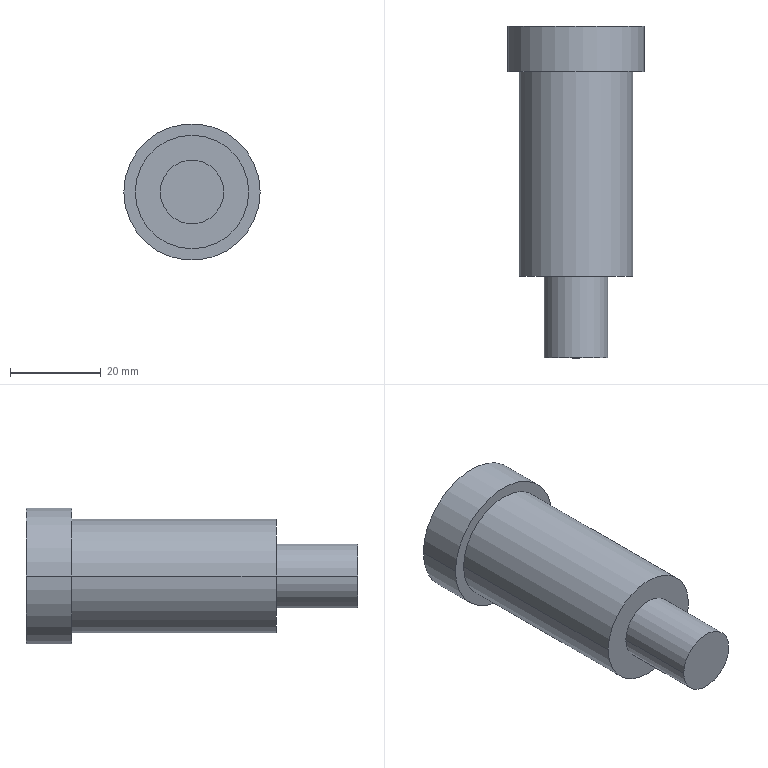Component | SolidWorks | FlipAxis-4 | 1 solid | 10 faces | box 30 x 73 x 30 mm | volume 31929 mm3 | cylinder 6 | plane 4 | commonest cylinder face diameters 14 x2 25 x2 30 x2 | material Plain Carbon Steel
build123d program:
from build123d import *

# Parameters (mm, degrees)
SKETCH1_R           = 15
BOSS_EXTRUDE1_DEPTH = 10
SKETCH2_R           = 12.5
BOSS_EXTRUDE2_DEPTH = 45
SKETCH3_R           = 7
BOSS_EXTRUDE3_DEPTH = 18


with BuildPart() as part:
    # Sketch1 → Boss-Extrude1 (new body)
    with BuildSketch(Plane.XY):
        Circle(SKETCH1_R)
    extrude(amount=BOSS_EXTRUDE1_DEPTH)

    # Sketch2 → Boss-Extrude2 (add)
    with BuildSketch(Plane.XY.offset(10)):
        with Locations(Location((0, 0, 0), (0, 0, 180))):
            Circle(SKETCH2_R)
    extrude(amount=BOSS_EXTRUDE2_DEPTH)

    # Sketch3 → Boss-Extrude3 (add)
    with BuildSketch(Plane.XY.offset(55)):
        Circle(SKETCH3_R)
    extrude(amount=BOSS_EXTRUDE3_DEPTH)


solid = part.part

# Placed as in the assembly
solid = solid.moved(Location((-864.885, -397.907, 1035.102), (90, 0, 0)))
STEP:
#1=COLOUR_RGB('',0.7922,0.8196,0.9333);
#2=FILL_AREA_STYLE_COLOUR('',#1);
#3=FILL_AREA_STYLE('',(#2));
#4=SURFACE_STYLE_FILL_AREA(#3);
#5=SURFACE_SIDE_STYLE('',(#4));
#6=SURFACE_STYLE_USAGE(.BOTH.,#5);
#7=PRESENTATION_STYLE_ASSIGNMENT((#6));
#8=CARTESIAN_POINT('',(-33.775,-18.54,40.752));
#9=VERTEX_POINT('',#8);
#10=CARTESIAN_POINT('',(-34.326,-18.54,40.752));
#11=VERTEX_POINT('',#10);
#12=CARTESIAN_POINT('',(-34.051,-18.54,40.752));
#13=DIRECTION('',(0.,-1.,0.));
#14=DIRECTION('',(1.,0.,0.));
#15=AXIS2_PLACEMENT_3D('',#12,#13,#14);
#16=CIRCLE('',#15,0.2756);
#17=EDGE_CURVE('',#9,#11,#16,.T.);
#18=ORIENTED_EDGE('',*,*,#17,.F.);
#19=CARTESIAN_POINT('',(-33.775,-17.831,40.752));
#20=VERTEX_POINT('',#19);
#21=CARTESIAN_POINT('',(-33.775,-18.54,40.752));
#22=DIRECTION('',(0.,1.,0.));
#23=VECTOR('',#22,39.37);
#24=LINE('',#21,#23);
#25=EDGE_CURVE('',#9,#20,#24,.T.);
#26=ORIENTED_EDGE('',*,*,#25,.T.);
#27=CARTESIAN_POINT('',(-34.326,-17.831,40.752));
#28=VERTEX_POINT('',#27);
#29=CARTESIAN_POINT('',(-34.051,-17.831,40.752));
#30=DIRECTION('',(0.,-1.,0.));
#31=DIRECTION('',(1.,0.,0.));
#32=AXIS2_PLACEMENT_3D('',#29,#30,#31);
#33=CIRCLE('',#32,0.2756);
#34=EDGE_CURVE('',#20,#28,#33,.T.);
#35=ORIENTED_EDGE('',*,*,#34,.T.);
#36=CARTESIAN_POINT('',(-34.326,-18.54,40.752));
#37=DIRECTION('',(0.,1.,0.));
#38=VECTOR('',#37,39.37);
#39=LINE('',#36,#38);
#40=EDGE_CURVE('',#11,#28,#39,.T.);
#41=ORIENTED_EDGE('',*,*,#40,.F.);
#42=EDGE_LOOP('',(#18,#26,#35,#41));
#43=FACE_OUTER_BOUND('',#42,.T.);
#44=CARTESIAN_POINT('',(-34.051,-18.54,40.752));
#45=DIRECTION('',(0.,1.,0.));
#46=DIRECTION('',(-1.,0.,0.));
#47=AXIS2_PLACEMENT_3D('',#44,#45,#46);
#48=CYLINDRICAL_SURFACE('',#47,0.2756);
#49=ADVANCED_FACE('',(#43),#48,.T.);
#50=CARTESIAN_POINT('',(-33.558,-17.831,40.752));
#51=VERTEX_POINT('',#50);
#52=CARTESIAN_POINT('',(-34.543,-17.831,40.752));
#53=VERTEX_POINT('',#52);
#54=CARTESIAN_POINT('',(-34.051,-17.831,40.752));
#55=DIRECTION('',(0.,-1.,0.));
#56=DIRECTION('',(1.,0.,0.));
#57=AXIS2_PLACEMENT_3D('',#54,#55,#56);
#58=CIRCLE('',#57,0.4921);
#59=EDGE_CURVE('',#51,#53,#58,.T.);
#60=ORIENTED_EDGE('',*,*,#59,.F.);
#61=CARTESIAN_POINT('',(-33.558,-16.059,40.752));
#62=VERTEX_POINT('',#61);
#63=CARTESIAN_POINT('',(-33.558,-17.831,40.752));
#64=DIRECTION('',(0.,1.,0.));
#65=VECTOR('',#64,39.37);
#66=LINE('',#63,#65);
#67=EDGE_CURVE('',#51,#62,#66,.T.);
#68=ORIENTED_EDGE('',*,*,#67,.T.);
#69=CARTESIAN_POINT('',(-34.543,-16.059,40.752));
#70=VERTEX_POINT('',#69);
#71=CARTESIAN_POINT('',(-34.051,-16.059,40.752));
#72=DIRECTION('',(0.,-1.,0.));
#73=DIRECTION('',(1.,0.,0.));
#74=AXIS2_PLACEMENT_3D('',#71,#72,#73);
#75=CIRCLE('',#74,0.4921);
#76=EDGE_CURVE('',#62,#70,#75,.T.);
#77=ORIENTED_EDGE('',*,*,#76,.T.);
#78=CARTESIAN_POINT('',(-34.543,-17.831,40.752));
#79=DIRECTION('',(0.,1.,0.));
#80=VECTOR('',#79,39.37);
#81=LINE('',#78,#80);
#82=EDGE_CURVE('',#53,#70,#81,.T.);
#83=ORIENTED_EDGE('',*,*,#82,.F.);
#84=EDGE_LOOP('',(#60,#68,#77,#83));
#85=FACE_OUTER_BOUND('',#84,.T.);
#86=CARTESIAN_POINT('',(-34.051,-17.831,40.752));
#87=DIRECTION('',(0.,1.,0.));
#88=DIRECTION('',(-1.,0.,0.));
#89=AXIS2_PLACEMENT_3D('',#86,#87,#88);
#90=CYLINDRICAL_SURFACE('',#89,0.4921);
#91=ADVANCED_FACE('',(#85),#90,.T.);
#92=CARTESIAN_POINT('',(-33.46,-16.059,40.752));
#93=VERTEX_POINT('',#92);
#94=CARTESIAN_POINT('',(-34.641,-16.059,40.752));
#95=VERTEX_POINT('',#94);
#96=CARTESIAN_POINT('',(-34.051,-16.059,40.752));
#97=DIRECTION('',(0.,-1.,0.));
#98=DIRECTION('',(1.,0.,0.));
#99=AXIS2_PLACEMENT_3D('',#96,#97,#98);
#100=CIRCLE('',#99,0.5906);
#101=EDGE_CURVE('',#93,#95,#100,.T.);
#102=ORIENTED_EDGE('',*,*,#101,.F.);
#103=CARTESIAN_POINT('',(-33.46,-15.666,40.752));
#104=VERTEX_POINT('',#103);
#105=CARTESIAN_POINT('',(-33.46,-16.059,40.752));
#106=DIRECTION('',(0.,1.,0.));
#107=VECTOR('',#106,39.37);
#108=LINE('',#105,#107);
#109=EDGE_CURVE('',#93,#104,#108,.T.);
#110=ORIENTED_EDGE('',*,*,#109,.T.);
#111=CARTESIAN_POINT('',(-34.641,-15.666,40.752));
#112=VERTEX_POINT('',#111);
#113=CARTESIAN_POINT('',(-34.051,-15.666,40.752));
#114=DIRECTION('',(0.,-1.,0.));
#115=DIRECTION('',(1.,0.,0.));
#116=AXIS2_PLACEMENT_3D('',#113,#114,#115);
#117=CIRCLE('',#116,0.5906);
#118=EDGE_CURVE('',#104,#112,#117,.T.);
#119=ORIENTED_EDGE('',*,*,#118,.T.);
#120=CARTESIAN_POINT('',(-34.641,-16.059,40.752));
#121=DIRECTION('',(0.,1.,0.));
#122=VECTOR('',#121,39.37);
#123=LINE('',#120,#122);
#124=EDGE_CURVE('',#95,#112,#123,.T.);
#125=ORIENTED_EDGE('',*,*,#124,.F.);
#126=EDGE_LOOP('',(#102,#110,#119,#125));
#127=FACE_OUTER_BOUND('',#126,.T.);
#128=CARTESIAN_POINT('',(-34.051,-16.059,40.752));
#129=DIRECTION('',(0.,1.,0.));
#130=DIRECTION('',(-1.,0.,0.));
#131=AXIS2_PLACEMENT_3D('',#128,#129,#130);
#132=CYLINDRICAL_SURFACE('',#131,0.5906);
#133=ADVANCED_FACE('',(#127),#132,.T.);
#134=CARTESIAN_POINT('',(-34.051,-17.831,40.752));
#135=DIRECTION('',(0.,-1.,0.));
#136=DIRECTION('',(1.,0.,0.));
#137=AXIS2_PLACEMENT_3D('',#134,#135,#136);
#138=CIRCLE('',#137,0.4921);
#139=EDGE_CURVE('',#53,#51,#138,.T.);
#140=ORIENTED_EDGE('',*,*,#139,.T.);
#141=ORIENTED_EDGE('',*,*,#59,.T.);
#142=EDGE_LOOP('',(#140,#141));
#143=FACE_OUTER_BOUND('',#142,.T.);
#144=CARTESIAN_POINT('',(-34.051,-17.831,40.752));
#145=DIRECTION('',(0.,-1.,0.));
#146=DIRECTION('',(1.,0.,0.));
#147=AXIS2_PLACEMENT_3D('',#144,#145,#146);
#148=CIRCLE('',#147,0.2756);
#149=EDGE_CURVE('',#28,#20,#148,.T.);
#150=ORIENTED_EDGE('',*,*,#149,.F.);
#151=ORIENTED_EDGE('',*,*,#34,.F.);
#152=EDGE_LOOP('',(#150,#151));
#153=FACE_BOUND('',#152,.T.);
#154=CARTESIAN_POINT('',(-34.051,-17.831,40.752));
#155=DIRECTION('',(0.,-1.,0.));
#156=DIRECTION('',(1.,0.,0.));
#157=AXIS2_PLACEMENT_3D('',#154,#155,#156);
#158=PLANE('',#157);
#159=ADVANCED_FACE('',(#143,#153),#158,.T.);
#160=CARTESIAN_POINT('',(-34.051,-16.059,40.752));
#161=DIRECTION('',(0.,-1.,0.));
#162=DIRECTION('',(1.,0.,0.));
#163=AXIS2_PLACEMENT_3D('',#160,#161,#162);
#164=CIRCLE('',#163,0.5906);
#165=EDGE_CURVE('',#95,#93,#164,.T.);
#166=ORIENTED_EDGE('',*,*,#165,.T.);
#167=ORIENTED_EDGE('',*,*,#101,.T.);
#168=EDGE_LOOP('',(#166,#167));
#169=FACE_OUTER_BOUND('',#168,.T.);
#170=CARTESIAN_POINT('',(-34.051,-16.059,40.752));
#171=DIRECTION('',(0.,-1.,0.));
#172=DIRECTION('',(1.,0.,0.));
#173=AXIS2_PLACEMENT_3D('',#170,#171,#172);
#174=CIRCLE('',#173,0.4921);
#175=EDGE_CURVE('',#70,#62,#174,.T.);
#176=ORIENTED_EDGE('',*,*,#175,.F.);
#177=ORIENTED_EDGE('',*,*,#76,.F.);
#178=EDGE_LOOP('',(#176,#177));
#179=FACE_BOUND('',#178,.T.);
#180=CARTESIAN_POINT('',(-34.051,-16.059,40.752));
#181=DIRECTION('',(0.,-1.,0.));
#182=DIRECTION('',(1.,0.,0.));
#183=AXIS2_PLACEMENT_3D('',#180,#181,#182);
#184=PLANE('',#183);
#185=ADVANCED_FACE('',(#169,#179),#184,.T.);
#186=ORIENTED_EDGE('',*,*,#109,.F.);
#187=ORIENTED_EDGE('',*,*,#165,.F.);
#188=ORIENTED_EDGE('',*,*,#124,.T.);
#189=CARTESIAN_POINT('',(-34.051,-15.666,40.752));
#190=DIRECTION('',(0.,-1.,0.));
#191=DIRECTION('',(1.,0.,0.));
#192=AXIS2_PLACEMENT_3D('',#189,#190,#191);
#193=CIRCLE('',#192,0.5906);
#194=EDGE_CURVE('',#112,#104,#193,.T.);
#195=ORIENTED_EDGE('',*,*,#194,.T.);
#196=EDGE_LOOP('',(#186,#187,#188,#195));
#197=FACE_OUTER_BOUND('',#196,.T.);
#198=CARTESIAN_POINT('',(-34.051,-16.059,40.752));
#199=DIRECTION('',(0.,1.,0.));
#200=DIRECTION('',(-1.,0.,0.));
#201=AXIS2_PLACEMENT_3D('',#198,#199,#200);
#202=CYLINDRICAL_SURFACE('',#201,0.5906);
#203=ADVANCED_FACE('',(#197),#202,.T.);
#204=ORIENTED_EDGE('',*,*,#194,.F.);
#205=ORIENTED_EDGE('',*,*,#118,.F.);
#206=EDGE_LOOP('',(#204,#205));
#207=FACE_OUTER_BOUND('',#206,.T.);
#208=CARTESIAN_POINT('',(-34.051,-15.666,40.752));
#209=DIRECTION('',(0.,-1.,0.));
#210=DIRECTION('',(1.,0.,0.));
#211=AXIS2_PLACEMENT_3D('',#208,#209,#210);
#212=PLANE('',#211);
#213=ADVANCED_FACE('',(#207),#212,.F.);
#214=ORIENTED_EDGE('',*,*,#67,.F.);
#215=ORIENTED_EDGE('',*,*,#139,.F.);
#216=ORIENTED_EDGE('',*,*,#82,.T.);
#217=ORIENTED_EDGE('',*,*,#175,.T.);
#218=EDGE_LOOP('',(#214,#215,#216,#217));
#219=FACE_OUTER_BOUND('',#218,.T.);
#220=CARTESIAN_POINT('',(-34.051,-17.831,40.752));
#221=DIRECTION('',(0.,1.,0.));
#222=DIRECTION('',(-1.,0.,0.));
#223=AXIS2_PLACEMENT_3D('',#220,#221,#222);
#224=CYLINDRICAL_SURFACE('',#223,0.4921);
#225=ADVANCED_FACE('',(#219),#224,.T.);
#226=ORIENTED_EDGE('',*,*,#25,.F.);
#227=CARTESIAN_POINT('',(-34.051,-18.54,40.752));
#228=DIRECTION('',(0.,-1.,0.));
#229=DIRECTION('',(1.,0.,0.));
#230=AXIS2_PLACEMENT_3D('',#227,#228,#229);
#231=CIRCLE('',#230,0.2756);
#232=EDGE_CURVE('',#11,#9,#231,.T.);
#233=ORIENTED_EDGE('',*,*,#232,.F.);
#234=ORIENTED_EDGE('',*,*,#40,.T.);
#235=ORIENTED_EDGE('',*,*,#149,.T.);
#236=EDGE_LOOP('',(#226,#233,#234,#235));
#237=FACE_OUTER_BOUND('',#236,.T.);
#238=CARTESIAN_POINT('',(-34.051,-18.54,40.752));
#239=DIRECTION('',(0.,1.,0.));
#240=DIRECTION('',(-1.,0.,0.));
#241=AXIS2_PLACEMENT_3D('',#238,#239,#240);
#242=CYLINDRICAL_SURFACE('',#241,0.2756);
#243=ADVANCED_FACE('',(#237),#242,.T.);
#244=ORIENTED_EDGE('',*,*,#232,.T.);
#245=ORIENTED_EDGE('',*,*,#17,.T.);
#246=EDGE_LOOP('',(#244,#245));
#247=FACE_OUTER_BOUND('',#246,.T.);
#248=CARTESIAN_POINT('',(-34.051,-18.54,40.752));
#249=DIRECTION('',(0.,-1.,0.));
#250=DIRECTION('',(1.,0.,0.));
#251=AXIS2_PLACEMENT_3D('',#248,#249,#250);
#252=PLANE('',#251);
#253=ADVANCED_FACE('',(#247),#252,.T.);
#254=CLOSED_SHELL('',(#49,#91,#133,#159,#185,#203,#213,#225,#243,#253));
#255=MANIFOLD_SOLID_BREP('',#254);
#256=STYLED_ITEM('',(#7),#255);
#257=PRESENTATION_LAYER_ASSIGNMENT('','',(#256));
#258=(LENGTH_UNIT()NAMED_UNIT(*)SI_UNIT($,.METRE.));
#259=LENGTH_MEASURE_WITH_UNIT(LENGTH_MEASURE(0.0254),#258);
#260=DIMENSIONAL_EXPONENTS(1.,0.,0.,0.,0.,0.,0.);
#261=(CONVERSION_BASED_UNIT('',#259)LENGTH_UNIT()NAMED_UNIT(#260));
#262=UNCERTAINTY_MEASURE_WITH_UNIT(LENGTH_MEASURE(0.00001),#261,'','');
#263=(NAMED_UNIT(*)PLANE_ANGLE_UNIT()SI_UNIT($,.RADIAN.));
#264=(NAMED_UNIT(*)SI_UNIT($,.STERADIAN.)SOLID_ANGLE_UNIT());
#265=(GEOMETRIC_REPRESENTATION_CONTEXT(3)GLOBAL_UNCERTAINTY_ASSIGNED_CONTEXT((#262))GLOBAL_UNIT_ASSIGNED_CONTEXT((#261,#263,#264))REPRESENTATION_CONTEXT('',''));
#266=MECHANICAL_DESIGN_GEOMETRIC_PRESENTATION_REPRESENTATION('',(#256),#265);
#267=CARTESIAN_POINT('',(0.,0.,0.));
#268=DIRECTION('',(0.,0.,1.));
#269=DIRECTION('',(1.,0.,0.));
#270=AXIS2_PLACEMENT_3D('',#267,#268,#269);
#271=(LENGTH_UNIT()NAMED_UNIT(*)SI_UNIT($,.METRE.));
#272=LENGTH_MEASURE_WITH_UNIT(LENGTH_MEASURE(0.0254),#271);
#273=DIMENSIONAL_EXPONENTS(1.,0.,0.,0.,0.,0.,0.);
#274=(CONVERSION_BASED_UNIT('',#272)LENGTH_UNIT()NAMED_UNIT(#273));
#275=UNCERTAINTY_MEASURE_WITH_UNIT(LENGTH_MEASURE(0.00001),#274,'','');
#276=(NAMED_UNIT(*)PLANE_ANGLE_UNIT()SI_UNIT($,.RADIAN.));
#277=(NAMED_UNIT(*)SI_UNIT($,.STERADIAN.)SOLID_ANGLE_UNIT());
#278=(GEOMETRIC_REPRESENTATION_CONTEXT(3)GLOBAL_UNCERTAINTY_ASSIGNED_CONTEXT((#275))GLOBAL_UNIT_ASSIGNED_CONTEXT((#274,#276,#277))REPRESENTATION_CONTEXT('',''));
#279=ADVANCED_BREP_SHAPE_REPRESENTATION('',(#255,#270),#278);